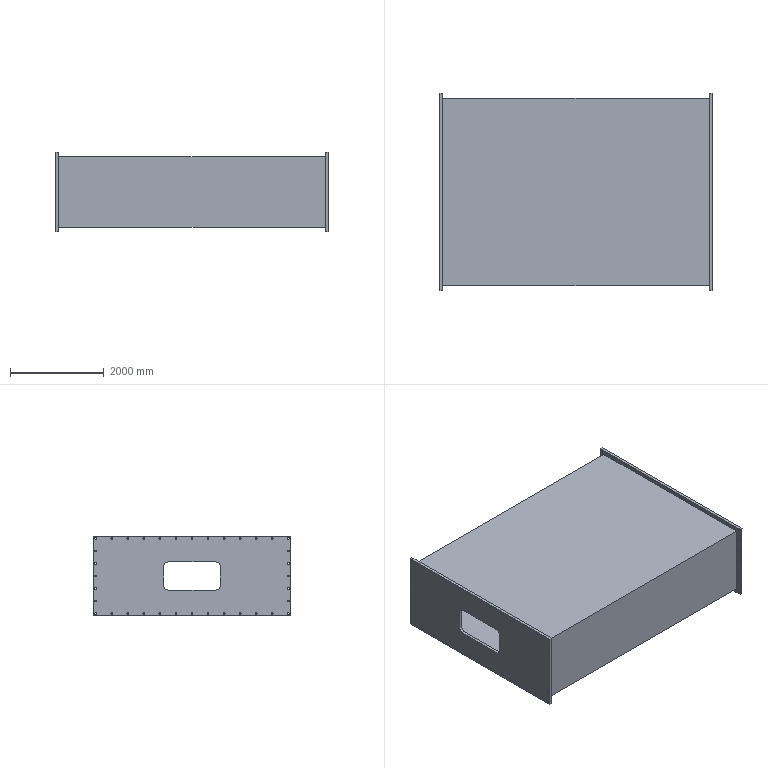Component | SolidWorks | EndBeam-1 | 1 solid | 224 faces | volume 3665797983 mm3 | cylinder 164 | plane 60 | commonest cylinder face diameters 40 x144 200 x20